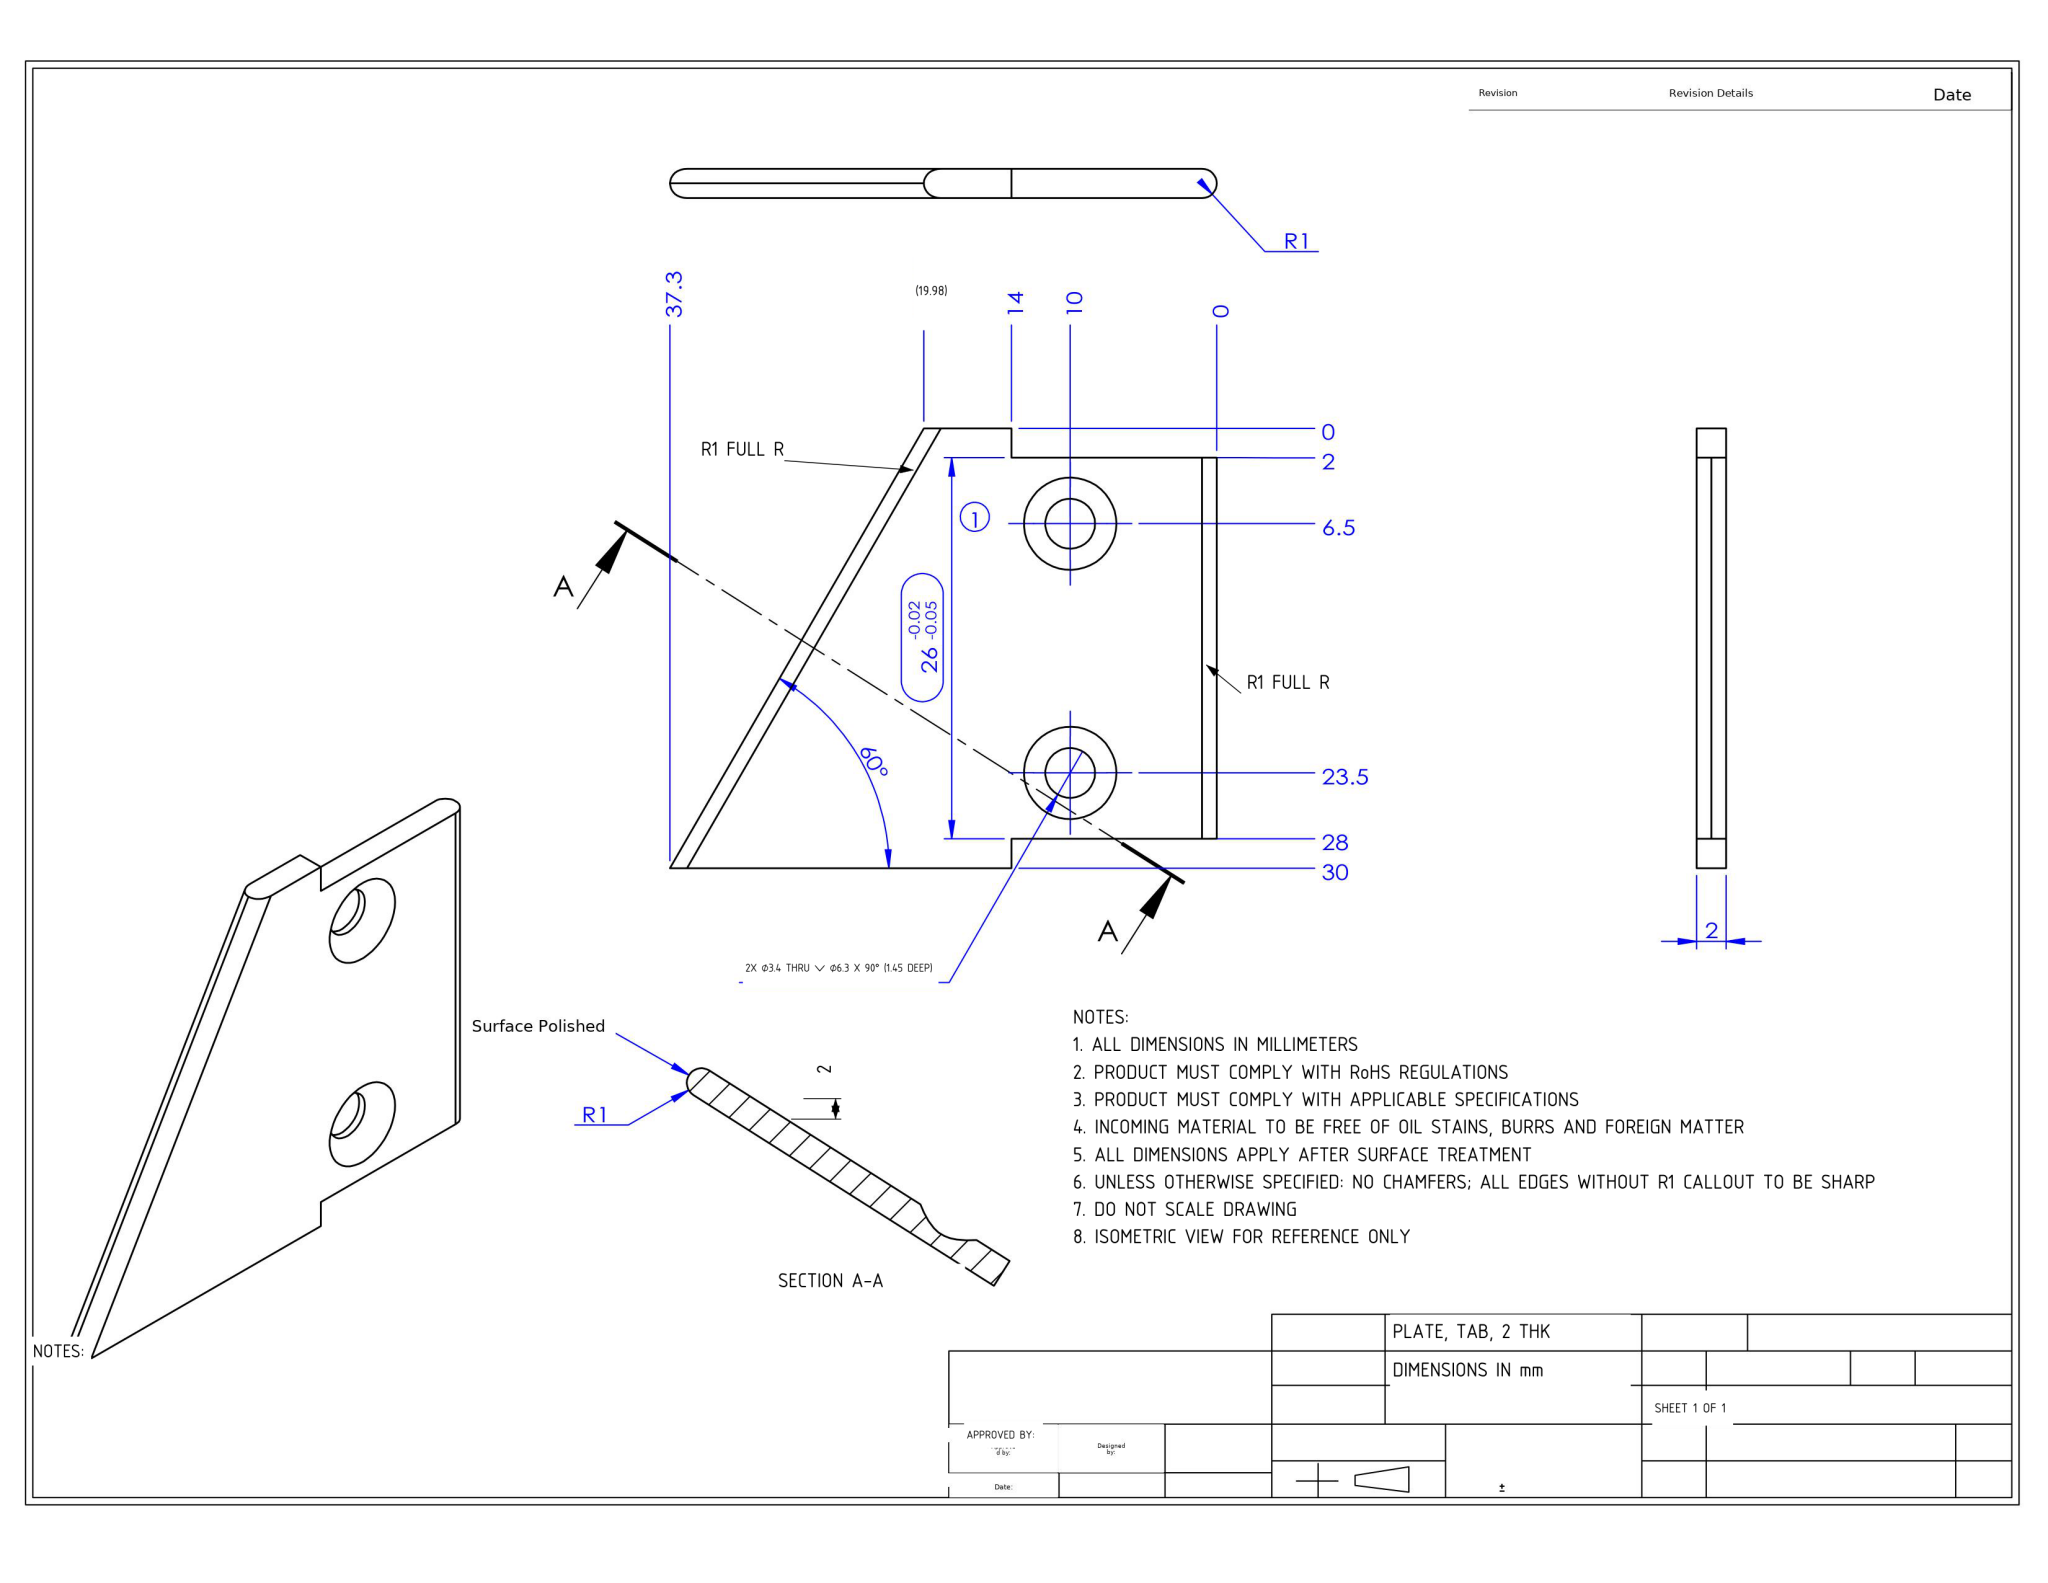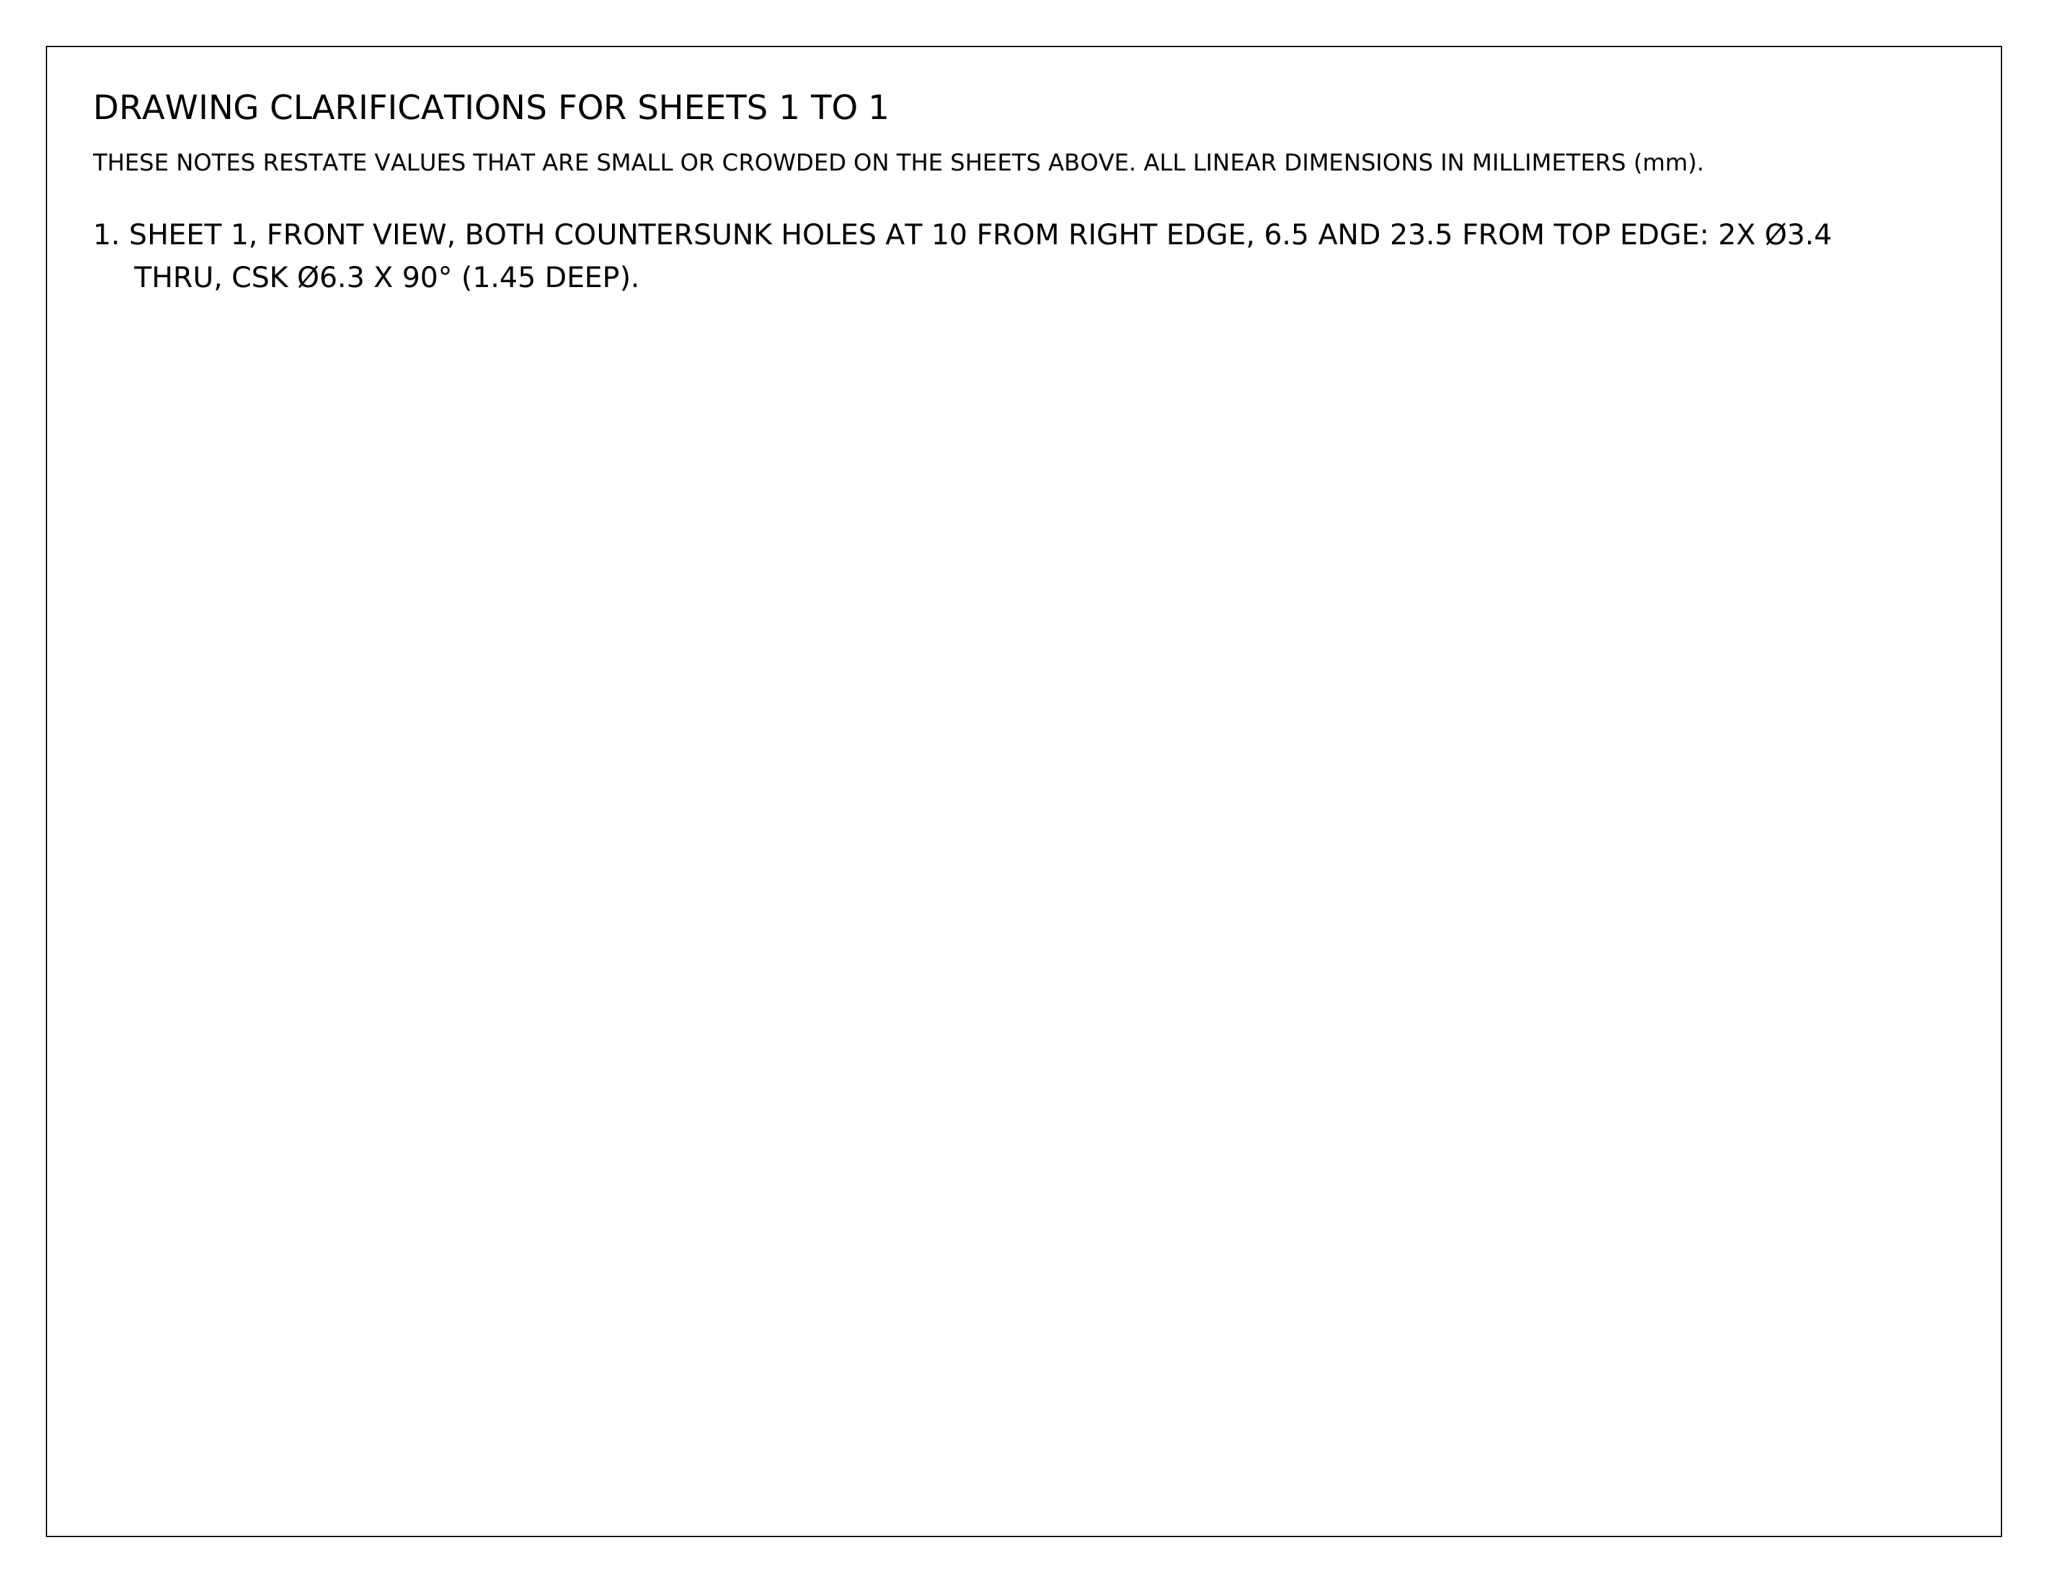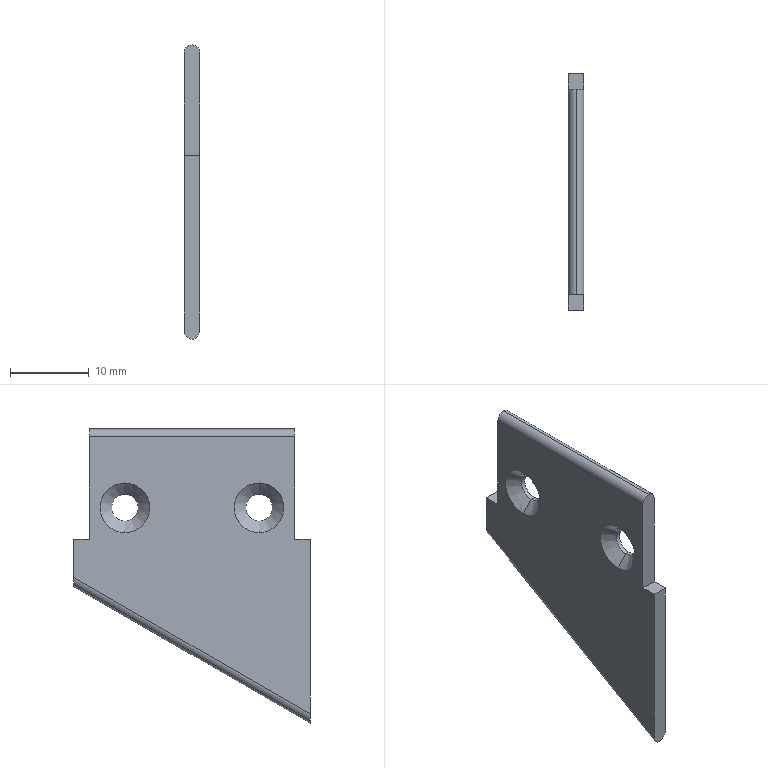Part | NX | mm | 1 solid | 20 faces | box 2 x 30 x 37.3 mm | volume 1515 mm3 | cylinder 8 | plane 8 | cone 4 | commonest cylinder face diameters 3.4 x4 2 x4
STEP:
#1=COLOUR_RGB('',0.8941,0.9137,0.9294);
#2=FILL_AREA_STYLE_COLOUR('',#1);
#3=FILL_AREA_STYLE('',(#2));
#4=SURFACE_STYLE_FILL_AREA(#3);
#5=SURFACE_SIDE_STYLE('',(#4));
#6=SURFACE_STYLE_USAGE(.BOTH.,#5);
#7=PRESENTATION_STYLE_ASSIGNMENT((#6));
#8=CARTESIAN_POINT('',(1.45,-8.5,9.95));
#9=VERTEX_POINT('',#8);
#10=CARTESIAN_POINT('',(1.45,-8.5,13.35));
#11=VERTEX_POINT('',#10);
#12=CARTESIAN_POINT('',(1.45,-8.5,11.65));
#13=DIRECTION('',(-1.,0.,0.));
#14=DIRECTION('',(0.,0.,1.));
#15=AXIS2_PLACEMENT_3D('',#12,#13,#14);
#16=CIRCLE('',#15,1.7);
#17=EDGE_CURVE('',#9,#11,#16,.T.);
#18=ORIENTED_EDGE('',*,*,#17,.F.);
#19=CARTESIAN_POINT('',(-0.,-8.5,8.5));
#20=VERTEX_POINT('',#19);
#21=CARTESIAN_POINT('',(-0.,-8.5,8.5));
#22=DIRECTION('',(-0.7071,0.,-0.7071));
#23=VECTOR('',#22,1000.);
#24=LINE('',#21,#23);
#25=EDGE_CURVE('',#9,#20,#24,.T.);
#26=ORIENTED_EDGE('',*,*,#25,.T.);
#27=CARTESIAN_POINT('',(-0.,-8.5,14.8));
#28=VERTEX_POINT('',#27);
#29=CARTESIAN_POINT('',(-0.,-8.5,11.65));
#30=DIRECTION('',(-1.,0.,0.));
#31=DIRECTION('',(0.,0.,1.));
#32=AXIS2_PLACEMENT_3D('',#29,#30,#31);
#33=CIRCLE('',#32,3.15);
#34=EDGE_CURVE('',#20,#28,#33,.T.);
#35=ORIENTED_EDGE('',*,*,#34,.T.);
#36=CARTESIAN_POINT('',(-0.,-8.5,14.8));
#37=DIRECTION('',(-0.7071,0.,0.7071));
#38=VECTOR('',#37,1000.);
#39=LINE('',#36,#38);
#40=EDGE_CURVE('',#11,#28,#39,.T.);
#41=ORIENTED_EDGE('',*,*,#40,.F.);
#42=EDGE_LOOP('',(#18,#26,#35,#41));
#43=FACE_OUTER_BOUND('',#42,.T.);
#44=CARTESIAN_POINT('',(-0.,-8.5,11.65));
#45=DIRECTION('',(-1.,0.,0.));
#46=DIRECTION('',(0.,0.,1.));
#47=AXIS2_PLACEMENT_3D('',#44,#45,#46);
#48=CONICAL_SURFACE('',#47,3.15,0.7854);
#49=ADVANCED_FACE('',(#43),#48,.F.);
#50=CARTESIAN_POINT('',(2.,-8.5,9.95));
#51=VERTEX_POINT('',#50);
#52=CARTESIAN_POINT('',(2.,-8.5,13.35));
#53=VERTEX_POINT('',#52);
#54=CARTESIAN_POINT('',(2.,-8.5,11.65));
#55=DIRECTION('',(-1.,0.,0.));
#56=DIRECTION('',(0.,0.,1.));
#57=AXIS2_PLACEMENT_3D('',#54,#55,#56);
#58=CIRCLE('',#57,1.7);
#59=EDGE_CURVE('',#51,#53,#58,.T.);
#60=ORIENTED_EDGE('',*,*,#59,.F.);
#61=CARTESIAN_POINT('',(0.,-8.5,9.95));
#62=DIRECTION('',(-1.,0.,0.));
#63=VECTOR('',#62,1000.);
#64=LINE('',#61,#63);
#65=EDGE_CURVE('',#51,#9,#64,.T.);
#66=ORIENTED_EDGE('',*,*,#65,.T.);
#67=ORIENTED_EDGE('',*,*,#17,.T.);
#68=CARTESIAN_POINT('',(0.,-8.5,13.35));
#69=DIRECTION('',(-1.,0.,0.));
#70=VECTOR('',#69,1000.);
#71=LINE('',#68,#70);
#72=EDGE_CURVE('',#53,#11,#71,.T.);
#73=ORIENTED_EDGE('',*,*,#72,.F.);
#74=EDGE_LOOP('',(#60,#66,#67,#73));
#75=FACE_OUTER_BOUND('',#74,.T.);
#76=CARTESIAN_POINT('',(0.,-8.5,11.65));
#77=DIRECTION('',(-1.,0.,0.));
#78=DIRECTION('',(0.,0.,1.));
#79=AXIS2_PLACEMENT_3D('',#76,#77,#78);
#80=CYLINDRICAL_SURFACE('',#79,1.7);
#81=ADVANCED_FACE('',(#75),#80,.F.);
#82=CARTESIAN_POINT('',(1.45,8.5,9.95));
#83=VERTEX_POINT('',#82);
#84=CARTESIAN_POINT('',(1.45,8.5,13.35));
#85=VERTEX_POINT('',#84);
#86=CARTESIAN_POINT('',(1.45,8.5,11.65));
#87=DIRECTION('',(-1.,0.,0.));
#88=DIRECTION('',(0.,0.,1.));
#89=AXIS2_PLACEMENT_3D('',#86,#87,#88);
#90=CIRCLE('',#89,1.7);
#91=EDGE_CURVE('',#83,#85,#90,.T.);
#92=ORIENTED_EDGE('',*,*,#91,.F.);
#93=CARTESIAN_POINT('',(-0.,8.5,8.5));
#94=VERTEX_POINT('',#93);
#95=CARTESIAN_POINT('',(-0.,8.5,8.5));
#96=DIRECTION('',(-0.7071,0.,-0.7071));
#97=VECTOR('',#96,1000.);
#98=LINE('',#95,#97);
#99=EDGE_CURVE('',#83,#94,#98,.T.);
#100=ORIENTED_EDGE('',*,*,#99,.T.);
#101=CARTESIAN_POINT('',(-0.,8.5,14.8));
#102=VERTEX_POINT('',#101);
#103=CARTESIAN_POINT('',(-0.,8.5,11.65));
#104=DIRECTION('',(-1.,0.,0.));
#105=DIRECTION('',(0.,0.,1.));
#106=AXIS2_PLACEMENT_3D('',#103,#104,#105);
#107=CIRCLE('',#106,3.15);
#108=EDGE_CURVE('',#94,#102,#107,.T.);
#109=ORIENTED_EDGE('',*,*,#108,.T.);
#110=CARTESIAN_POINT('',(-0.,8.5,14.8));
#111=DIRECTION('',(-0.7071,0.,0.7071));
#112=VECTOR('',#111,1000.);
#113=LINE('',#110,#112);
#114=EDGE_CURVE('',#85,#102,#113,.T.);
#115=ORIENTED_EDGE('',*,*,#114,.F.);
#116=EDGE_LOOP('',(#92,#100,#109,#115));
#117=FACE_OUTER_BOUND('',#116,.T.);
#118=CARTESIAN_POINT('',(-0.,8.5,11.65));
#119=DIRECTION('',(-1.,0.,0.));
#120=DIRECTION('',(0.,0.,1.));
#121=AXIS2_PLACEMENT_3D('',#118,#119,#120);
#122=CONICAL_SURFACE('',#121,3.15,0.7854);
#123=ADVANCED_FACE('',(#117),#122,.F.);
#124=CARTESIAN_POINT('',(2.,8.5,9.95));
#125=VERTEX_POINT('',#124);
#126=CARTESIAN_POINT('',(2.,8.5,13.35));
#127=VERTEX_POINT('',#126);
#128=CARTESIAN_POINT('',(2.,8.5,11.65));
#129=DIRECTION('',(-1.,0.,0.));
#130=DIRECTION('',(0.,0.,1.));
#131=AXIS2_PLACEMENT_3D('',#128,#129,#130);
#132=CIRCLE('',#131,1.7);
#133=EDGE_CURVE('',#125,#127,#132,.T.);
#134=ORIENTED_EDGE('',*,*,#133,.F.);
#135=CARTESIAN_POINT('',(0.,8.5,9.95));
#136=DIRECTION('',(-1.,0.,0.));
#137=VECTOR('',#136,1000.);
#138=LINE('',#135,#137);
#139=EDGE_CURVE('',#125,#83,#138,.T.);
#140=ORIENTED_EDGE('',*,*,#139,.T.);
#141=ORIENTED_EDGE('',*,*,#91,.T.);
#142=CARTESIAN_POINT('',(0.,8.5,13.35));
#143=DIRECTION('',(-1.,0.,0.));
#144=VECTOR('',#143,1000.);
#145=LINE('',#142,#144);
#146=EDGE_CURVE('',#127,#85,#145,.T.);
#147=ORIENTED_EDGE('',*,*,#146,.F.);
#148=EDGE_LOOP('',(#134,#140,#141,#147));
#149=FACE_OUTER_BOUND('',#148,.T.);
#150=CARTESIAN_POINT('',(0.,8.5,11.65));
#151=DIRECTION('',(-1.,0.,0.));
#152=DIRECTION('',(0.,0.,1.));
#153=AXIS2_PLACEMENT_3D('',#150,#151,#152);
#154=CYLINDRICAL_SURFACE('',#153,1.7);
#155=ADVANCED_FACE('',(#149),#154,.F.);
#156=CARTESIAN_POINT('',(2.,-15.,7.65));
#157=VERTEX_POINT('',#156);
#158=CARTESIAN_POINT('',(2.,-15.,-14.495));
#159=VERTEX_POINT('',#158);
#160=CARTESIAN_POINT('',(2.,-15.,-15.65));
#161=DIRECTION('',(0.,0.,-1.));
#162=VECTOR('',#161,1000.);
#163=LINE('',#160,#162);
#164=EDGE_CURVE('',#157,#159,#163,.T.);
#165=ORIENTED_EDGE('',*,*,#164,.F.);
#166=CARTESIAN_POINT('',(0.,-15.,7.65));
#167=VERTEX_POINT('',#166);
#168=CARTESIAN_POINT('',(0.,-15.,7.65));
#169=DIRECTION('',(1.,0.,0.));
#170=VECTOR('',#169,1000.);
#171=LINE('',#168,#170);
#172=EDGE_CURVE('',#167,#157,#171,.T.);
#173=ORIENTED_EDGE('',*,*,#172,.F.);
#174=CARTESIAN_POINT('',(0.,-15.,-14.495));
#175=VERTEX_POINT('',#174);
#176=CARTESIAN_POINT('',(0.,-15.,-15.65));
#177=DIRECTION('',(0.,0.,-1.));
#178=VECTOR('',#177,1000.);
#179=LINE('',#176,#178);
#180=EDGE_CURVE('',#167,#175,#179,.T.);
#181=ORIENTED_EDGE('',*,*,#180,.T.);
#182=CARTESIAN_POINT('',(1.,-15.,-15.65));
#183=VERTEX_POINT('',#182);
#184=CARTESIAN_POINT('',(0.,-15.,-14.495));
#185=CARTESIAN_POINT('',(-0.,-15.,-15.172));
#186=CARTESIAN_POINT('',(0.4142,-15.,-15.65));
#187=CARTESIAN_POINT('',(1.,-15.,-15.65));
#188=(BOUNDED_CURVE()B_SPLINE_CURVE(3,(#184,#185,#186,#187),.UNSPECIFIED.,.F.,.F.)B_SPLINE_CURVE_WITH_KNOTS((4,4),(4.712,6.283),.UNSPECIFIED.)CURVE()GEOMETRIC_REPRESENTATION_ITEM()RATIONAL_B_SPLINE_CURVE((1.,0.8047,0.8047,1.))REPRESENTATION_ITEM(''));
#189=EDGE_CURVE('',#175,#183,#188,.T.);
#190=ORIENTED_EDGE('',*,*,#189,.T.);
#191=CARTESIAN_POINT('',(1.,-15.,-15.65));
#192=CARTESIAN_POINT('',(1.586,-15.,-15.65));
#193=CARTESIAN_POINT('',(2.,-15.,-15.172));
#194=CARTESIAN_POINT('',(2.,-15.,-14.495));
#195=(BOUNDED_CURVE()B_SPLINE_CURVE(3,(#191,#192,#193,#194),.UNSPECIFIED.,.F.,.T.)B_SPLINE_CURVE_WITH_KNOTS((4,4),(3.142,4.712),.UNSPECIFIED.)CURVE()GEOMETRIC_REPRESENTATION_ITEM()RATIONAL_B_SPLINE_CURVE((1.,0.8047,0.8047,1.))REPRESENTATION_ITEM(''));
#196=EDGE_CURVE('',#183,#159,#195,.T.);
#197=ORIENTED_EDGE('',*,*,#196,.T.);
#198=EDGE_LOOP('',(#165,#173,#181,#190,#197));
#199=FACE_OUTER_BOUND('',#198,.T.);
#200=CARTESIAN_POINT('',(2.,-15.,-15.65));
#201=DIRECTION('',(0.,1.,0.));
#202=DIRECTION('',(0.,-0.,1.));
#203=AXIS2_PLACEMENT_3D('',#200,#201,#202);
#204=PLANE('',#203);
#205=ADVANCED_FACE('',(#199),#204,.F.);
#206=CARTESIAN_POINT('',(0.,15.,2.825));
#207=VERTEX_POINT('',#206);
#208=CARTESIAN_POINT('',(0.,15.,7.65));
#209=VERTEX_POINT('',#208);
#210=CARTESIAN_POINT('',(0.,15.,-15.65));
#211=DIRECTION('',(0.,-0.,1.));
#212=VECTOR('',#211,1000.);
#213=LINE('',#210,#212);
#214=EDGE_CURVE('',#207,#209,#213,.T.);
#215=ORIENTED_EDGE('',*,*,#214,.T.);
#216=CARTESIAN_POINT('',(2.,15.,7.65));
#217=VERTEX_POINT('',#216);
#218=CARTESIAN_POINT('',(0.,15.,7.65));
#219=DIRECTION('',(1.,0.,0.));
#220=VECTOR('',#219,1000.);
#221=LINE('',#218,#220);
#222=EDGE_CURVE('',#209,#217,#221,.T.);
#223=ORIENTED_EDGE('',*,*,#222,.T.);
#224=CARTESIAN_POINT('',(2.,15.,2.825));
#225=VERTEX_POINT('',#224);
#226=CARTESIAN_POINT('',(2.,15.,-15.65));
#227=DIRECTION('',(0.,-0.,1.));
#228=VECTOR('',#227,1000.);
#229=LINE('',#226,#228);
#230=EDGE_CURVE('',#225,#217,#229,.T.);
#231=ORIENTED_EDGE('',*,*,#230,.F.);
#232=CARTESIAN_POINT('',(1.,15.,1.671));
#233=VERTEX_POINT('',#232);
#234=CARTESIAN_POINT('',(2.,15.,2.825));
#235=CARTESIAN_POINT('',(2.,15.,2.149));
#236=CARTESIAN_POINT('',(1.586,15.,1.671));
#237=CARTESIAN_POINT('',(1.,15.,1.671));
#238=(BOUNDED_CURVE()B_SPLINE_CURVE(3,(#234,#235,#236,#237),.UNSPECIFIED.,.F.,.T.)B_SPLINE_CURVE_WITH_KNOTS((4,4),(1.571,3.142),.UNSPECIFIED.)CURVE()GEOMETRIC_REPRESENTATION_ITEM()RATIONAL_B_SPLINE_CURVE((1.,0.8047,0.8047,1.))REPRESENTATION_ITEM(''));
#239=EDGE_CURVE('',#225,#233,#238,.T.);
#240=ORIENTED_EDGE('',*,*,#239,.T.);
#241=CARTESIAN_POINT('',(1.,15.,1.671));
#242=CARTESIAN_POINT('',(0.4142,15.,1.671));
#243=CARTESIAN_POINT('',(-0.,15.,2.149));
#244=CARTESIAN_POINT('',(0.,15.,2.825));
#245=(BOUNDED_CURVE()B_SPLINE_CURVE(3,(#241,#242,#243,#244),.UNSPECIFIED.,.F.,.T.)B_SPLINE_CURVE_WITH_KNOTS((4,4),(0.,1.571),.UNSPECIFIED.)CURVE()GEOMETRIC_REPRESENTATION_ITEM()RATIONAL_B_SPLINE_CURVE((1.,0.8047,0.8047,1.))REPRESENTATION_ITEM(''));
#246=EDGE_CURVE('',#233,#207,#245,.T.);
#247=ORIENTED_EDGE('',*,*,#246,.T.);
#248=EDGE_LOOP('',(#215,#223,#231,#240,#247));
#249=FACE_OUTER_BOUND('',#248,.T.);
#250=CARTESIAN_POINT('',(2.,15.,-15.65));
#251=DIRECTION('',(0.,-1.,-0.));
#252=DIRECTION('',(0.,0.,-1.));
#253=AXIS2_PLACEMENT_3D('',#250,#251,#252);
#254=PLANE('',#253);
#255=ADVANCED_FACE('',(#249),#254,.F.);
#256=CARTESIAN_POINT('',(2.,-8.5,11.65));
#257=DIRECTION('',(-1.,0.,0.));
#258=DIRECTION('',(0.,0.,1.));
#259=AXIS2_PLACEMENT_3D('',#256,#257,#258);
#260=CIRCLE('',#259,1.7);
#261=EDGE_CURVE('',#53,#51,#260,.T.);
#262=ORIENTED_EDGE('',*,*,#261,.T.);
#263=ORIENTED_EDGE('',*,*,#59,.T.);
#264=EDGE_LOOP('',(#262,#263));
#265=FACE_BOUND('',#264,.T.);
#266=CARTESIAN_POINT('',(2.,8.5,11.65));
#267=DIRECTION('',(-1.,0.,0.));
#268=DIRECTION('',(0.,0.,1.));
#269=AXIS2_PLACEMENT_3D('',#266,#267,#268);
#270=CIRCLE('',#269,1.7);
#271=EDGE_CURVE('',#127,#125,#270,.T.);
#272=ORIENTED_EDGE('',*,*,#271,.T.);
#273=ORIENTED_EDGE('',*,*,#133,.T.);
#274=EDGE_LOOP('',(#272,#273));
#275=FACE_BOUND('',#274,.T.);
#276=CARTESIAN_POINT('',(2.,13.,20.65));
#277=VERTEX_POINT('',#276);
#278=CARTESIAN_POINT('',(2.,13.,7.65));
#279=VERTEX_POINT('',#278);
#280=CARTESIAN_POINT('',(2.,13.,15.65));
#281=DIRECTION('',(0.,0.,-1.));
#282=VECTOR('',#281,1000.);
#283=LINE('',#280,#282);
#284=EDGE_CURVE('',#277,#279,#283,.T.);
#285=ORIENTED_EDGE('',*,*,#284,.F.);
#286=CARTESIAN_POINT('',(2.,-13.,20.65));
#287=VERTEX_POINT('',#286);
#288=CARTESIAN_POINT('',(2.,-13.,20.65));
#289=DIRECTION('',(0.,-1.,0.));
#290=VECTOR('',#289,1000.);
#291=LINE('',#288,#290);
#292=EDGE_CURVE('',#277,#287,#291,.T.);
#293=ORIENTED_EDGE('',*,*,#292,.T.);
#294=CARTESIAN_POINT('',(2.,-13.,7.65));
#295=VERTEX_POINT('',#294);
#296=CARTESIAN_POINT('',(2.,-13.,15.65));
#297=DIRECTION('',(0.,0.,1.));
#298=VECTOR('',#297,1000.);
#299=LINE('',#296,#298);
#300=EDGE_CURVE('',#295,#287,#299,.T.);
#301=ORIENTED_EDGE('',*,*,#300,.F.);
#302=CARTESIAN_POINT('',(2.,-15.,7.65));
#303=DIRECTION('',(0.,1.,-0.));
#304=VECTOR('',#303,1000.);
#305=LINE('',#302,#304);
#306=EDGE_CURVE('',#157,#295,#305,.T.);
#307=ORIENTED_EDGE('',*,*,#306,.F.);
#308=ORIENTED_EDGE('',*,*,#164,.T.);
#309=CARTESIAN_POINT('',(2.,14.5,2.537));
#310=DIRECTION('',(0.,0.866,0.5));
#311=VECTOR('',#310,1000.);
#312=LINE('',#309,#311);
#313=EDGE_CURVE('',#159,#225,#312,.T.);
#314=ORIENTED_EDGE('',*,*,#313,.T.);
#315=ORIENTED_EDGE('',*,*,#230,.T.);
#316=CARTESIAN_POINT('',(2.,15.,7.65));
#317=DIRECTION('',(0.,1.,0.));
#318=VECTOR('',#317,1000.);
#319=LINE('',#316,#318);
#320=EDGE_CURVE('',#279,#217,#319,.T.);
#321=ORIENTED_EDGE('',*,*,#320,.F.);
#322=EDGE_LOOP('',(#285,#293,#301,#307,#308,#314,#315,#321));
#323=FACE_OUTER_BOUND('',#322,.T.);
#324=CARTESIAN_POINT('',(2.,0.,0.));
#325=DIRECTION('',(1.,0.,0.));
#326=DIRECTION('',(0.,0.,-1.));
#327=AXIS2_PLACEMENT_3D('',#324,#325,#326);
#328=PLANE('',#327);
#329=ADVANCED_FACE('',(#265,#275,#323),#328,.T.);
#330=CARTESIAN_POINT('',(-0.,-8.5,11.65));
#331=DIRECTION('',(-1.,0.,0.));
#332=DIRECTION('',(0.,0.,1.));
#333=AXIS2_PLACEMENT_3D('',#330,#331,#332);
#334=CIRCLE('',#333,3.15);
#335=EDGE_CURVE('',#28,#20,#334,.T.);
#336=ORIENTED_EDGE('',*,*,#335,.F.);
#337=ORIENTED_EDGE('',*,*,#34,.F.);
#338=EDGE_LOOP('',(#336,#337));
#339=FACE_BOUND('',#338,.T.);
#340=CARTESIAN_POINT('',(-0.,8.5,11.65));
#341=DIRECTION('',(-1.,0.,0.));
#342=DIRECTION('',(0.,0.,1.));
#343=AXIS2_PLACEMENT_3D('',#340,#341,#342);
#344=CIRCLE('',#343,3.15);
#345=EDGE_CURVE('',#102,#94,#344,.T.);
#346=ORIENTED_EDGE('',*,*,#345,.F.);
#347=ORIENTED_EDGE('',*,*,#108,.F.);
#348=EDGE_LOOP('',(#346,#347));
#349=FACE_BOUND('',#348,.T.);
#350=CARTESIAN_POINT('',(0.,-13.,7.65));
#351=VERTEX_POINT('',#350);
#352=CARTESIAN_POINT('',(0.,-13.,20.65));
#353=VERTEX_POINT('',#352);
#354=CARTESIAN_POINT('',(0.,-13.,15.65));
#355=DIRECTION('',(0.,0.,1.));
#356=VECTOR('',#355,1000.);
#357=LINE('',#354,#356);
#358=EDGE_CURVE('',#351,#353,#357,.T.);
#359=ORIENTED_EDGE('',*,*,#358,.T.);
#360=CARTESIAN_POINT('',(0.,13.,20.65));
#361=VERTEX_POINT('',#360);
#362=CARTESIAN_POINT('',(0.,0.,20.65));
#363=DIRECTION('',(0.,1.,0.));
#364=VECTOR('',#363,1000.);
#365=LINE('',#362,#364);
#366=EDGE_CURVE('',#353,#361,#365,.T.);
#367=ORIENTED_EDGE('',*,*,#366,.T.);
#368=CARTESIAN_POINT('',(0.,13.,7.65));
#369=VERTEX_POINT('',#368);
#370=CARTESIAN_POINT('',(0.,13.,15.65));
#371=DIRECTION('',(0.,0.,-1.));
#372=VECTOR('',#371,1000.);
#373=LINE('',#370,#372);
#374=EDGE_CURVE('',#361,#369,#373,.T.);
#375=ORIENTED_EDGE('',*,*,#374,.T.);
#376=CARTESIAN_POINT('',(0.,15.,7.65));
#377=DIRECTION('',(0.,1.,0.));
#378=VECTOR('',#377,1000.);
#379=LINE('',#376,#378);
#380=EDGE_CURVE('',#369,#209,#379,.T.);
#381=ORIENTED_EDGE('',*,*,#380,.T.);
#382=ORIENTED_EDGE('',*,*,#214,.F.);
#383=CARTESIAN_POINT('',(0.,2.527,-4.376));
#384=DIRECTION('',(0.,-0.866,-0.5));
#385=VECTOR('',#384,1000.);
#386=LINE('',#383,#385);
#387=EDGE_CURVE('',#207,#175,#386,.T.);
#388=ORIENTED_EDGE('',*,*,#387,.T.);
#389=ORIENTED_EDGE('',*,*,#180,.F.);
#390=CARTESIAN_POINT('',(0.,-15.,7.65));
#391=DIRECTION('',(0.,1.,-0.));
#392=VECTOR('',#391,1000.);
#393=LINE('',#390,#392);
#394=EDGE_CURVE('',#167,#351,#393,.T.);
#395=ORIENTED_EDGE('',*,*,#394,.T.);
#396=EDGE_LOOP('',(#359,#367,#375,#381,#382,#388,#389,#395));
#397=FACE_OUTER_BOUND('',#396,.T.);
#398=CARTESIAN_POINT('',(0.,0.,0.));
#399=DIRECTION('',(1.,0.,0.));
#400=DIRECTION('',(0.,0.,-1.));
#401=AXIS2_PLACEMENT_3D('',#398,#399,#400);
#402=PLANE('',#401);
#403=ADVANCED_FACE('',(#339,#349,#397),#402,.F.);
#404=CARTESIAN_POINT('',(1.,-15.,-15.65));
#405=DIRECTION('',(0.,-0.866,-0.5));
#406=VECTOR('',#405,1000.);
#407=LINE('',#404,#406);
#408=EDGE_CURVE('',#233,#183,#407,.T.);
#409=ORIENTED_EDGE('',*,*,#408,.F.);
#410=ORIENTED_EDGE('',*,*,#239,.F.);
#411=ORIENTED_EDGE('',*,*,#313,.F.);
#412=ORIENTED_EDGE('',*,*,#196,.F.);
#413=EDGE_LOOP('',(#409,#410,#411,#412));
#414=FACE_OUTER_BOUND('',#413,.T.);
#415=CARTESIAN_POINT('',(1.,-15.5,-14.784));
#416=DIRECTION('',(0.,0.866,0.5));
#417=DIRECTION('',(0.,-0.5,0.866));
#418=AXIS2_PLACEMENT_3D('',#415,#416,#417);
#419=CYLINDRICAL_SURFACE('',#418,1.);
#420=ADVANCED_FACE('',(#414),#419,.T.);
#421=ORIENTED_EDGE('',*,*,#246,.F.);
#422=ORIENTED_EDGE('',*,*,#408,.T.);
#423=ORIENTED_EDGE('',*,*,#189,.F.);
#424=ORIENTED_EDGE('',*,*,#387,.F.);
#425=EDGE_LOOP('',(#421,#422,#423,#424));
#426=FACE_OUTER_BOUND('',#425,.T.);
#427=CARTESIAN_POINT('',(1.,2.527,-4.376));
#428=DIRECTION('',(0.,-0.866,-0.5));
#429=DIRECTION('',(0.,0.5,-0.866));
#430=AXIS2_PLACEMENT_3D('',#427,#428,#429);
#431=CYLINDRICAL_SURFACE('',#430,1.);
#432=ADVANCED_FACE('',(#426),#431,.T.);
#433=ORIENTED_EDGE('',*,*,#320,.T.);
#434=ORIENTED_EDGE('',*,*,#222,.F.);
#435=ORIENTED_EDGE('',*,*,#380,.F.);
#436=CARTESIAN_POINT('',(0.,13.,7.65));
#437=DIRECTION('',(1.,0.,0.));
#438=VECTOR('',#437,1000.);
#439=LINE('',#436,#438);
#440=EDGE_CURVE('',#369,#279,#439,.T.);
#441=ORIENTED_EDGE('',*,*,#440,.T.);
#442=EDGE_LOOP('',(#433,#434,#435,#441));
#443=FACE_OUTER_BOUND('',#442,.T.);
#444=CARTESIAN_POINT('',(0.,15.,7.65));
#445=DIRECTION('',(0.,0.,-1.));
#446=DIRECTION('',(0.,1.,0.));
#447=AXIS2_PLACEMENT_3D('',#444,#445,#446);
#448=PLANE('',#447);
#449=ADVANCED_FACE('',(#443),#448,.F.);
#450=CARTESIAN_POINT('',(1.,13.,21.65));
#451=VERTEX_POINT('',#450);
#452=CARTESIAN_POINT('',(1.,13.,20.65));
#453=DIRECTION('',(0.,1.,0.));
#454=DIRECTION('',(0.,0.,-1.));
#455=AXIS2_PLACEMENT_3D('',#452,#453,#454);
#456=CIRCLE('',#455,1.);
#457=EDGE_CURVE('',#361,#451,#456,.T.);
#458=ORIENTED_EDGE('',*,*,#457,.T.);
#459=CARTESIAN_POINT('',(1.,13.,20.65));
#460=DIRECTION('',(0.,1.,0.));
#461=DIRECTION('',(0.,0.,-1.));
#462=AXIS2_PLACEMENT_3D('',#459,#460,#461);
#463=CIRCLE('',#462,1.);
#464=EDGE_CURVE('',#451,#277,#463,.T.);
#465=ORIENTED_EDGE('',*,*,#464,.T.);
#466=ORIENTED_EDGE('',*,*,#284,.T.);
#467=ORIENTED_EDGE('',*,*,#440,.F.);
#468=ORIENTED_EDGE('',*,*,#374,.F.);
#469=EDGE_LOOP('',(#458,#465,#466,#467,#468));
#470=FACE_OUTER_BOUND('',#469,.T.);
#471=CARTESIAN_POINT('',(0.,13.,15.65));
#472=DIRECTION('',(0.,-1.,0.));
#473=DIRECTION('',(0.,0.,-1.));
#474=AXIS2_PLACEMENT_3D('',#471,#472,#473);
#475=PLANE('',#474);
#476=ADVANCED_FACE('',(#470),#475,.F.);
#477=ORIENTED_EDGE('',*,*,#300,.T.);
#478=CARTESIAN_POINT('',(1.,-13.,21.65));
#479=VERTEX_POINT('',#478);
#480=CARTESIAN_POINT('',(1.,-13.,20.65));
#481=DIRECTION('',(0.,-1.,0.));
#482=DIRECTION('',(0.,0.,1.));
#483=AXIS2_PLACEMENT_3D('',#480,#481,#482);
#484=CIRCLE('',#483,1.);
#485=EDGE_CURVE('',#287,#479,#484,.T.);
#486=ORIENTED_EDGE('',*,*,#485,.T.);
#487=CARTESIAN_POINT('',(1.,-13.,20.65));
#488=DIRECTION('',(0.,-1.,0.));
#489=DIRECTION('',(0.,0.,1.));
#490=AXIS2_PLACEMENT_3D('',#487,#488,#489);
#491=CIRCLE('',#490,1.);
#492=EDGE_CURVE('',#479,#353,#491,.T.);
#493=ORIENTED_EDGE('',*,*,#492,.T.);
#494=ORIENTED_EDGE('',*,*,#358,.F.);
#495=CARTESIAN_POINT('',(0.,-13.,7.65));
#496=DIRECTION('',(1.,0.,0.));
#497=VECTOR('',#496,1000.);
#498=LINE('',#495,#497);
#499=EDGE_CURVE('',#351,#295,#498,.T.);
#500=ORIENTED_EDGE('',*,*,#499,.T.);
#501=EDGE_LOOP('',(#477,#486,#493,#494,#500));
#502=FACE_OUTER_BOUND('',#501,.T.);
#503=CARTESIAN_POINT('',(0.,-13.,15.65));
#504=DIRECTION('',(0.,1.,0.));
#505=DIRECTION('',(0.,0.,1.));
#506=AXIS2_PLACEMENT_3D('',#503,#504,#505);
#507=PLANE('',#506);
#508=ADVANCED_FACE('',(#502),#507,.F.);
#509=ORIENTED_EDGE('',*,*,#306,.T.);
#510=ORIENTED_EDGE('',*,*,#499,.F.);
#511=ORIENTED_EDGE('',*,*,#394,.F.);
#512=ORIENTED_EDGE('',*,*,#172,.T.);
#513=EDGE_LOOP('',(#509,#510,#511,#512));
#514=FACE_OUTER_BOUND('',#513,.T.);
#515=CARTESIAN_POINT('',(0.,-15.,7.65));
#516=DIRECTION('',(0.,-0.,-1.));
#517=DIRECTION('',(0.,1.,-0.));
#518=AXIS2_PLACEMENT_3D('',#515,#516,#517);
#519=PLANE('',#518);
#520=ADVANCED_FACE('',(#514),#519,.F.);
#521=ORIENTED_EDGE('',*,*,#139,.F.);
#522=ORIENTED_EDGE('',*,*,#271,.F.);
#523=ORIENTED_EDGE('',*,*,#146,.T.);
#524=CARTESIAN_POINT('',(1.45,8.5,11.65));
#525=DIRECTION('',(-1.,0.,0.));
#526=DIRECTION('',(0.,0.,1.));
#527=AXIS2_PLACEMENT_3D('',#524,#525,#526);
#528=CIRCLE('',#527,1.7);
#529=EDGE_CURVE('',#85,#83,#528,.T.);
#530=ORIENTED_EDGE('',*,*,#529,.T.);
#531=EDGE_LOOP('',(#521,#522,#523,#530));
#532=FACE_OUTER_BOUND('',#531,.T.);
#533=CARTESIAN_POINT('',(0.,8.5,11.65));
#534=DIRECTION('',(-1.,0.,0.));
#535=DIRECTION('',(0.,0.,1.));
#536=AXIS2_PLACEMENT_3D('',#533,#534,#535);
#537=CYLINDRICAL_SURFACE('',#536,1.7);
#538=ADVANCED_FACE('',(#532),#537,.F.);
#539=ORIENTED_EDGE('',*,*,#99,.F.);
#540=ORIENTED_EDGE('',*,*,#529,.F.);
#541=ORIENTED_EDGE('',*,*,#114,.T.);
#542=ORIENTED_EDGE('',*,*,#345,.T.);
#543=EDGE_LOOP('',(#539,#540,#541,#542));
#544=FACE_OUTER_BOUND('',#543,.T.);
#545=CARTESIAN_POINT('',(-0.,8.5,11.65));
#546=DIRECTION('',(-1.,0.,0.));
#547=DIRECTION('',(0.,0.,1.));
#548=AXIS2_PLACEMENT_3D('',#545,#546,#547);
#549=CONICAL_SURFACE('',#548,3.15,0.7854);
#550=ADVANCED_FACE('',(#544),#549,.F.);
#551=ORIENTED_EDGE('',*,*,#65,.F.);
#552=ORIENTED_EDGE('',*,*,#261,.F.);
#553=ORIENTED_EDGE('',*,*,#72,.T.);
#554=CARTESIAN_POINT('',(1.45,-8.5,11.65));
#555=DIRECTION('',(-1.,0.,0.));
#556=DIRECTION('',(0.,0.,1.));
#557=AXIS2_PLACEMENT_3D('',#554,#555,#556);
#558=CIRCLE('',#557,1.7);
#559=EDGE_CURVE('',#11,#9,#558,.T.);
#560=ORIENTED_EDGE('',*,*,#559,.T.);
#561=EDGE_LOOP('',(#551,#552,#553,#560));
#562=FACE_OUTER_BOUND('',#561,.T.);
#563=CARTESIAN_POINT('',(0.,-8.5,11.65));
#564=DIRECTION('',(-1.,0.,0.));
#565=DIRECTION('',(0.,0.,1.));
#566=AXIS2_PLACEMENT_3D('',#563,#564,#565);
#567=CYLINDRICAL_SURFACE('',#566,1.7);
#568=ADVANCED_FACE('',(#562),#567,.F.);
#569=ORIENTED_EDGE('',*,*,#25,.F.);
#570=ORIENTED_EDGE('',*,*,#559,.F.);
#571=ORIENTED_EDGE('',*,*,#40,.T.);
#572=ORIENTED_EDGE('',*,*,#335,.T.);
#573=EDGE_LOOP('',(#569,#570,#571,#572));
#574=FACE_OUTER_BOUND('',#573,.T.);
#575=CARTESIAN_POINT('',(-0.,-8.5,11.65));
#576=DIRECTION('',(-1.,0.,0.));
#577=DIRECTION('',(0.,0.,1.));
#578=AXIS2_PLACEMENT_3D('',#575,#576,#577);
#579=CONICAL_SURFACE('',#578,3.15,0.7854);
#580=ADVANCED_FACE('',(#574),#579,.F.);
#581=CARTESIAN_POINT('',(1.,-15.,21.65));
#582=DIRECTION('',(0.,-1.,0.));
#583=VECTOR('',#582,1000.);
#584=LINE('',#581,#583);
#585=EDGE_CURVE('',#451,#479,#584,.T.);
#586=ORIENTED_EDGE('',*,*,#585,.F.);
#587=ORIENTED_EDGE('',*,*,#457,.F.);
#588=ORIENTED_EDGE('',*,*,#366,.F.);
#589=ORIENTED_EDGE('',*,*,#492,.F.);
#590=EDGE_LOOP('',(#586,#587,#588,#589));
#591=FACE_OUTER_BOUND('',#590,.T.);
#592=CARTESIAN_POINT('',(1.,-15.,20.65));
#593=DIRECTION('',(0.,-1.,0.));
#594=DIRECTION('',(0.,0.,-1.));
#595=AXIS2_PLACEMENT_3D('',#592,#593,#594);
#596=CYLINDRICAL_SURFACE('',#595,1.);
#597=ADVANCED_FACE('',(#591),#596,.T.);
#598=ORIENTED_EDGE('',*,*,#464,.F.);
#599=ORIENTED_EDGE('',*,*,#585,.T.);
#600=ORIENTED_EDGE('',*,*,#485,.F.);
#601=ORIENTED_EDGE('',*,*,#292,.F.);
#602=EDGE_LOOP('',(#598,#599,#600,#601));
#603=FACE_OUTER_BOUND('',#602,.T.);
#604=CARTESIAN_POINT('',(1.,0.,20.65));
#605=DIRECTION('',(0.,1.,0.));
#606=DIRECTION('',(0.,0.,1.));
#607=AXIS2_PLACEMENT_3D('',#604,#605,#606);
#608=CYLINDRICAL_SURFACE('',#607,1.);
#609=ADVANCED_FACE('',(#603),#608,.T.);
#610=CLOSED_SHELL('',(#49,#81,#123,#155,#205,#255,#329,#403,#420,#432,#449,#476,#508,#520,#538,#550,#568,#580,#597,#609));
#611=MANIFOLD_SOLID_BREP('',#610);
#612=CARTESIAN_POINT('',(0.,0.,0.));
#613=DIRECTION('',(0.,0.,1.));
#614=DIRECTION('',(1.,0.,0.));
#615=AXIS2_PLACEMENT_3D('',#612,#613,#614);
#616=(LENGTH_UNIT()NAMED_UNIT(*)SI_UNIT(.MILLI.,.METRE.));
#617=UNCERTAINTY_MEASURE_WITH_UNIT(LENGTH_MEASURE(0.00001),#616,'','');
#618=(NAMED_UNIT(*)PLANE_ANGLE_UNIT()SI_UNIT($,.RADIAN.));
#619=(NAMED_UNIT(*)SI_UNIT($,.STERADIAN.)SOLID_ANGLE_UNIT());
#620=(GEOMETRIC_REPRESENTATION_CONTEXT(3)GLOBAL_UNCERTAINTY_ASSIGNED_CONTEXT((#617))GLOBAL_UNIT_ASSIGNED_CONTEXT((#616,#618,#619))REPRESENTATION_CONTEXT('',''));
#621=ADVANCED_BREP_SHAPE_REPRESENTATION('',(#611,#615),#620);
#622=STYLED_ITEM('',(#7),#621);
#623=(LENGTH_UNIT()NAMED_UNIT(*)SI_UNIT(.MILLI.,.METRE.));
#624=UNCERTAINTY_MEASURE_WITH_UNIT(LENGTH_MEASURE(0.00001),#623,'','');
#625=(NAMED_UNIT(*)PLANE_ANGLE_UNIT()SI_UNIT($,.RADIAN.));
#626=(NAMED_UNIT(*)SI_UNIT($,.STERADIAN.)SOLID_ANGLE_UNIT());
#627=(GEOMETRIC_REPRESENTATION_CONTEXT(3)GLOBAL_UNCERTAINTY_ASSIGNED_CONTEXT((#624))GLOBAL_UNIT_ASSIGNED_CONTEXT((#623,#625,#626))REPRESENTATION_CONTEXT('',''));
#628=MECHANICAL_DESIGN_GEOMETRIC_PRESENTATION_REPRESENTATION('',(#622),#627);
#629=COLOUR_RGB('',0.8941,0.9137,0.9294);
#630=FILL_AREA_STYLE_COLOUR('',#629);
#631=FILL_AREA_STYLE('',(#630));
#632=SURFACE_STYLE_FILL_AREA(#631);
#633=SURFACE_SIDE_STYLE('',(#632));
#634=SURFACE_STYLE_USAGE(.BOTH.,#633);
#635=PRESENTATION_STYLE_ASSIGNMENT((#634));
#636=STYLED_ITEM('',(#635),#611);
#637=PRESENTATION_LAYER_ASSIGNMENT('','',(#636));
#638=(LENGTH_UNIT()NAMED_UNIT(*)SI_UNIT(.MILLI.,.METRE.));
#639=UNCERTAINTY_MEASURE_WITH_UNIT(LENGTH_MEASURE(0.00001),#638,'','');
#640=(NAMED_UNIT(*)PLANE_ANGLE_UNIT()SI_UNIT($,.RADIAN.));
#641=(NAMED_UNIT(*)SI_UNIT($,.STERADIAN.)SOLID_ANGLE_UNIT());
#642=(GEOMETRIC_REPRESENTATION_CONTEXT(3)GLOBAL_UNCERTAINTY_ASSIGNED_CONTEXT((#639))GLOBAL_UNIT_ASSIGNED_CONTEXT((#638,#640,#641))REPRESENTATION_CONTEXT('',''));
#643=MECHANICAL_DESIGN_GEOMETRIC_PRESENTATION_REPRESENTATION('',(#636),#642);
#644=PRESENTATION_LAYER_ASSIGNMENT('','',(#622));